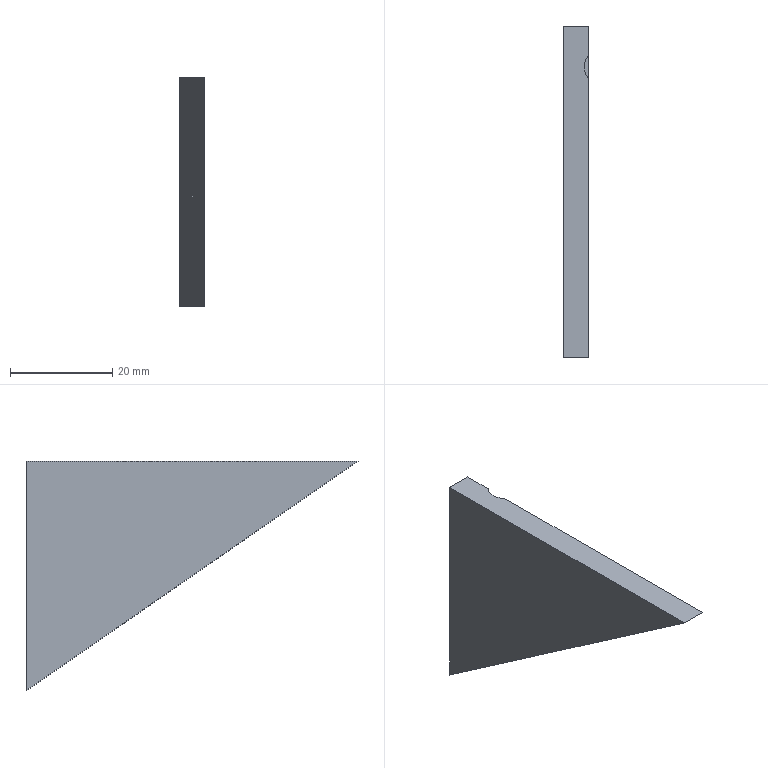Component | NX | FIXED_PLATE_14 | 1 solid | 7 faces | box 5 x 65 x 45 mm | volume 7284 mm3 | plane 6 | cylinder 1 | commonest cylinder face diameters 6.8 x1
STEP:
#1=CARTESIAN_POINT('',(0.,0.,0.));
#2=DIRECTION('',(0.,0.,1.));
#3=DIRECTION('',(1.,0.,0.));
#4=AXIS2_PLACEMENT_3D('',#1,#2,#3);
#5=CARTESIAN_POINT('',(1339.254,1356.,781.574));
#6=VERTEX_POINT('',#5);
#7=CARTESIAN_POINT('',(1339.254,1421.,736.574));
#8=VERTEX_POINT('',#7);
#9=CARTESIAN_POINT('',(1339.254,1356.,781.574));
#10=DIRECTION('',(0.,0.8222,-0.5692));
#11=VECTOR('',#10,1.);
#12=LINE('',#9,#11);
#13=CARTESIAN_POINT('',(1334.254,1356.,781.574));
#14=DIRECTION('',(0.,-0.5692,-0.8222));
#15=DIRECTION('',(0.,0.8222,-0.5692));
#16=AXIS2_PLACEMENT_3D('',#13,#14,#15);
#17=PLANE('',#16);
#18=CARTESIAN_POINT('',(0.,5.));
#19=DIRECTION('',(1.,0.));
#20=VECTOR('',#19,1.);
#21=LINE('',#18,#20);
#22=(GEOMETRIC_REPRESENTATION_CONTEXT(2)PARAMETRIC_REPRESENTATION_CONTEXT()REPRESENTATION_CONTEXT('',''));
#23=DEFINITIONAL_REPRESENTATION('',(#21),#22);
#24=PCURVE('',#17,#23);
#25=CARTESIAN_POINT('',(1339.254,0.,0.));
#26=DIRECTION('',(1.,0.,0.));
#27=DIRECTION('',(0.,0.,-1.));
#28=AXIS2_PLACEMENT_3D('',#25,#26,#27);
#29=PLANE('',#28);
#30=CARTESIAN_POINT('',(-781.574,1356.));
#31=DIRECTION('',(0.5692,0.8222));
#32=VECTOR('',#31,1.);
#33=LINE('',#30,#32);
#34=(GEOMETRIC_REPRESENTATION_CONTEXT(2)PARAMETRIC_REPRESENTATION_CONTEXT()REPRESENTATION_CONTEXT('',''));
#35=DEFINITIONAL_REPRESENTATION('',(#33),#34);
#36=PCURVE('',#29,#35);
#37=SURFACE_CURVE('',#12,(#24,#36),.PCURVE_S1.);
#38=EDGE_CURVE('',#6,#8,#37,.T.);
#39=ORIENTED_EDGE('',*,*,#38,.F.);
#40=CARTESIAN_POINT('',(1334.254,1356.,781.574));
#41=VERTEX_POINT('',#40);
#42=CARTESIAN_POINT('',(1334.254,1356.,781.574));
#43=DIRECTION('',(1.,0.,0.));
#44=VECTOR('',#43,1.);
#45=LINE('',#42,#44);
#46=CARTESIAN_POINT('',(0.,0.));
#47=DIRECTION('',(0.,1.));
#48=VECTOR('',#47,1.);
#49=LINE('',#46,#48);
#50=(GEOMETRIC_REPRESENTATION_CONTEXT(2)PARAMETRIC_REPRESENTATION_CONTEXT()REPRESENTATION_CONTEXT('',''));
#51=DEFINITIONAL_REPRESENTATION('',(#49),#50);
#52=PCURVE('',#17,#51);
#53=CARTESIAN_POINT('',(1334.254,1421.,781.574));
#54=DIRECTION('',(0.,0.,1.));
#55=DIRECTION('',(1.,0.,0.));
#56=AXIS2_PLACEMENT_3D('',#53,#54,#55);
#57=PLANE('',#56);
#58=CARTESIAN_POINT('',(0.,-65.));
#59=DIRECTION('',(1.,0.));
#60=VECTOR('',#59,1.);
#61=LINE('',#58,#60);
#62=(GEOMETRIC_REPRESENTATION_CONTEXT(2)PARAMETRIC_REPRESENTATION_CONTEXT()REPRESENTATION_CONTEXT('',''));
#63=DEFINITIONAL_REPRESENTATION('',(#61),#62);
#64=PCURVE('',#57,#63);
#65=SURFACE_CURVE('',#45,(#52,#64),.PCURVE_S1.);
#66=EDGE_CURVE('',#41,#6,#65,.T.);
#67=ORIENTED_EDGE('',*,*,#66,.F.);
#68=CARTESIAN_POINT('',(1334.254,1421.,736.574));
#69=VERTEX_POINT('',#68);
#70=CARTESIAN_POINT('',(1334.254,1356.,781.574));
#71=DIRECTION('',(0.,0.8222,-0.5692));
#72=VECTOR('',#71,1.);
#73=LINE('',#70,#72);
#74=CARTESIAN_POINT('',(0.,0.));
#75=DIRECTION('',(1.,0.));
#76=VECTOR('',#75,1.);
#77=LINE('',#74,#76);
#78=(GEOMETRIC_REPRESENTATION_CONTEXT(2)PARAMETRIC_REPRESENTATION_CONTEXT()REPRESENTATION_CONTEXT('',''));
#79=DEFINITIONAL_REPRESENTATION('',(#77),#78);
#80=PCURVE('',#17,#79);
#81=CARTESIAN_POINT('',(1334.254,0.,0.));
#82=DIRECTION('',(1.,0.,0.));
#83=DIRECTION('',(0.,0.,-1.));
#84=AXIS2_PLACEMENT_3D('',#81,#82,#83);
#85=PLANE('',#84);
#86=CARTESIAN_POINT('',(-781.574,1356.));
#87=DIRECTION('',(0.5692,0.8222));
#88=VECTOR('',#87,1.);
#89=LINE('',#86,#88);
#90=(GEOMETRIC_REPRESENTATION_CONTEXT(2)PARAMETRIC_REPRESENTATION_CONTEXT()REPRESENTATION_CONTEXT('',''));
#91=DEFINITIONAL_REPRESENTATION('',(#89),#90);
#92=PCURVE('',#85,#91);
#93=SURFACE_CURVE('',#73,(#80,#92),.PCURVE_S1.);
#94=EDGE_CURVE('',#41,#69,#93,.T.);
#95=ORIENTED_EDGE('',*,*,#94,.T.);
#96=CARTESIAN_POINT('',(1334.254,1421.,736.574));
#97=DIRECTION('',(1.,0.,0.));
#98=VECTOR('',#97,1.);
#99=LINE('',#96,#98);
#100=CARTESIAN_POINT('',(79.057,0.));
#101=DIRECTION('',(0.,1.));
#102=VECTOR('',#101,1.);
#103=LINE('',#100,#102);
#104=(GEOMETRIC_REPRESENTATION_CONTEXT(2)PARAMETRIC_REPRESENTATION_CONTEXT()REPRESENTATION_CONTEXT('',''));
#105=DEFINITIONAL_REPRESENTATION('',(#103),#104);
#106=PCURVE('',#17,#105);
#107=CARTESIAN_POINT('',(1334.254,1421.,736.574));
#108=DIRECTION('',(0.,1.,0.));
#109=DIRECTION('',(0.,0.,1.));
#110=AXIS2_PLACEMENT_3D('',#107,#108,#109);
#111=PLANE('',#110);
#112=CARTESIAN_POINT('',(0.,0.));
#113=DIRECTION('',(0.,1.));
#114=VECTOR('',#113,1.);
#115=LINE('',#112,#114);
#116=(GEOMETRIC_REPRESENTATION_CONTEXT(2)PARAMETRIC_REPRESENTATION_CONTEXT()REPRESENTATION_CONTEXT('',''));
#117=DEFINITIONAL_REPRESENTATION('',(#115),#116);
#118=PCURVE('',#111,#117);
#119=SURFACE_CURVE('',#99,(#106,#118),.PCURVE_S1.);
#120=EDGE_CURVE('',#69,#8,#119,.T.);
#121=ORIENTED_EDGE('',*,*,#120,.T.);
#122=EDGE_LOOP('',(#39,#67,#95,#121));
#123=FACE_BOUND('',#122,.T.);
#124=ADVANCED_FACE('',(#123),#17,.T.);
#125=CARTESIAN_POINT('',(1339.254,1421.,781.574));
#126=VERTEX_POINT('',#125);
#127=CARTESIAN_POINT('',(1339.254,1421.,736.574));
#128=DIRECTION('',(0.,0.,1.));
#129=VECTOR('',#128,1.);
#130=LINE('',#127,#129);
#131=CARTESIAN_POINT('',(0.,5.));
#132=DIRECTION('',(1.,0.));
#133=VECTOR('',#132,1.);
#134=LINE('',#131,#133);
#135=(GEOMETRIC_REPRESENTATION_CONTEXT(2)PARAMETRIC_REPRESENTATION_CONTEXT()REPRESENTATION_CONTEXT('',''));
#136=DEFINITIONAL_REPRESENTATION('',(#134),#135);
#137=PCURVE('',#111,#136);
#138=CARTESIAN_POINT('',(-736.574,1421.));
#139=DIRECTION('',(-1.,0.));
#140=VECTOR('',#139,1.);
#141=LINE('',#138,#140);
#142=(GEOMETRIC_REPRESENTATION_CONTEXT(2)PARAMETRIC_REPRESENTATION_CONTEXT()REPRESENTATION_CONTEXT('',''));
#143=DEFINITIONAL_REPRESENTATION('',(#141),#142);
#144=PCURVE('',#29,#143);
#145=SURFACE_CURVE('',#130,(#137,#144),.PCURVE_S1.);
#146=EDGE_CURVE('',#8,#126,#145,.T.);
#147=ORIENTED_EDGE('',*,*,#146,.F.);
#148=ORIENTED_EDGE('',*,*,#120,.F.);
#149=CARTESIAN_POINT('',(1334.254,1421.,781.574));
#150=VERTEX_POINT('',#149);
#151=CARTESIAN_POINT('',(1334.254,1421.,736.574));
#152=DIRECTION('',(0.,0.,1.));
#153=VECTOR('',#152,1.);
#154=LINE('',#151,#153);
#155=CARTESIAN_POINT('',(0.,0.));
#156=DIRECTION('',(1.,0.));
#157=VECTOR('',#156,1.);
#158=LINE('',#155,#157);
#159=(GEOMETRIC_REPRESENTATION_CONTEXT(2)PARAMETRIC_REPRESENTATION_CONTEXT()REPRESENTATION_CONTEXT('',''));
#160=DEFINITIONAL_REPRESENTATION('',(#158),#159);
#161=PCURVE('',#111,#160);
#162=CARTESIAN_POINT('',(-736.574,1421.));
#163=DIRECTION('',(-1.,0.));
#164=VECTOR('',#163,1.);
#165=LINE('',#162,#164);
#166=(GEOMETRIC_REPRESENTATION_CONTEXT(2)PARAMETRIC_REPRESENTATION_CONTEXT()REPRESENTATION_CONTEXT('',''));
#167=DEFINITIONAL_REPRESENTATION('',(#165),#166);
#168=PCURVE('',#85,#167);
#169=SURFACE_CURVE('',#154,(#161,#168),.PCURVE_S1.);
#170=EDGE_CURVE('',#69,#150,#169,.T.);
#171=ORIENTED_EDGE('',*,*,#170,.T.);
#172=CARTESIAN_POINT('',(1334.254,1421.,781.574));
#173=DIRECTION('',(1.,0.,0.));
#174=VECTOR('',#173,1.);
#175=LINE('',#172,#174);
#176=CARTESIAN_POINT('',(45.,0.));
#177=DIRECTION('',(0.,1.));
#178=VECTOR('',#177,1.);
#179=LINE('',#176,#178);
#180=(GEOMETRIC_REPRESENTATION_CONTEXT(2)PARAMETRIC_REPRESENTATION_CONTEXT()REPRESENTATION_CONTEXT('',''));
#181=DEFINITIONAL_REPRESENTATION('',(#179),#180);
#182=PCURVE('',#111,#181);
#183=CARTESIAN_POINT('',(0.,0.));
#184=DIRECTION('',(1.,0.));
#185=VECTOR('',#184,1.);
#186=LINE('',#183,#185);
#187=(GEOMETRIC_REPRESENTATION_CONTEXT(2)PARAMETRIC_REPRESENTATION_CONTEXT()REPRESENTATION_CONTEXT('',''));
#188=DEFINITIONAL_REPRESENTATION('',(#186),#187);
#189=PCURVE('',#57,#188);
#190=SURFACE_CURVE('',#175,(#182,#189),.PCURVE_S1.);
#191=EDGE_CURVE('',#150,#126,#190,.T.);
#192=ORIENTED_EDGE('',*,*,#191,.T.);
#193=EDGE_LOOP('',(#147,#148,#171,#192));
#194=FACE_BOUND('',#193,.T.);
#195=ADVANCED_FACE('',(#194),#111,.T.);
#196=CARTESIAN_POINT('',(1339.254,1415.304,781.574));
#197=VERTEX_POINT('',#196);
#198=CARTESIAN_POINT('',(1339.254,1410.696,781.574));
#199=VERTEX_POINT('',#198);
#200=CARTESIAN_POINT('',(1341.754,1413.,781.574));
#201=DIRECTION('',(0.,0.,1.));
#202=DIRECTION('',(0.,1.,0.));
#203=AXIS2_PLACEMENT_3D('',#200,#201,#202);
#204=CIRCLE('',#203,3.4);
#205=CARTESIAN_POINT('',(7.5,-8.));
#206=DIRECTION('',(0.,1.));
#207=AXIS2_PLACEMENT_2D('',#205,#206);
#208=CIRCLE('',#207,3.4);
#209=(GEOMETRIC_REPRESENTATION_CONTEXT(2)PARAMETRIC_REPRESENTATION_CONTEXT()REPRESENTATION_CONTEXT('',''));
#210=DEFINITIONAL_REPRESENTATION('',(#208),#209);
#211=PCURVE('',#57,#210);
#212=CARTESIAN_POINT('',(1341.754,1413.,771.574));
#213=DIRECTION('',(0.,0.,1.));
#214=DIRECTION('',(1.,0.,0.));
#215=AXIS2_PLACEMENT_3D('',#212,#213,#214);
#216=CYLINDRICAL_SURFACE('',#215,3.4);
#217=CARTESIAN_POINT('',(1.571,10.));
#218=DIRECTION('',(1.,0.));
#219=VECTOR('',#218,1.);
#220=LINE('',#217,#219);
#221=(GEOMETRIC_REPRESENTATION_CONTEXT(2)PARAMETRIC_REPRESENTATION_CONTEXT()REPRESENTATION_CONTEXT('',''));
#222=DEFINITIONAL_REPRESENTATION('',(#220),#221);
#223=PCURVE('',#216,#222);
#224=SURFACE_CURVE('',#204,(#211,#223),.PCURVE_S1.);
#225=EDGE_CURVE('',#197,#199,#224,.T.);
#226=ORIENTED_EDGE('',*,*,#225,.F.);
#227=CARTESIAN_POINT('',(1339.254,1421.,781.574));
#228=DIRECTION('',(0.,-1.,0.));
#229=VECTOR('',#228,1.);
#230=LINE('',#227,#229);
#231=CARTESIAN_POINT('',(5.,0.));
#232=DIRECTION('',(0.,-1.));
#233=VECTOR('',#232,1.);
#234=LINE('',#231,#233);
#235=(GEOMETRIC_REPRESENTATION_CONTEXT(2)PARAMETRIC_REPRESENTATION_CONTEXT()REPRESENTATION_CONTEXT('',''));
#236=DEFINITIONAL_REPRESENTATION('',(#234),#235);
#237=PCURVE('',#57,#236);
#238=CARTESIAN_POINT('',(-781.574,1421.));
#239=DIRECTION('',(0.,-1.));
#240=VECTOR('',#239,1.);
#241=LINE('',#238,#240);
#242=(GEOMETRIC_REPRESENTATION_CONTEXT(2)PARAMETRIC_REPRESENTATION_CONTEXT()REPRESENTATION_CONTEXT('',''));
#243=DEFINITIONAL_REPRESENTATION('',(#241),#242);
#244=PCURVE('',#29,#243);
#245=SURFACE_CURVE('',#230,(#237,#244),.PCURVE_S1.);
#246=EDGE_CURVE('',#126,#197,#245,.T.);
#247=ORIENTED_EDGE('',*,*,#246,.F.);
#248=ORIENTED_EDGE('',*,*,#191,.F.);
#249=CARTESIAN_POINT('',(1334.254,1421.,781.574));
#250=DIRECTION('',(0.,-1.,0.));
#251=VECTOR('',#250,1.);
#252=LINE('',#249,#251);
#253=CARTESIAN_POINT('',(0.,0.));
#254=DIRECTION('',(0.,-1.));
#255=VECTOR('',#254,1.);
#256=LINE('',#253,#255);
#257=(GEOMETRIC_REPRESENTATION_CONTEXT(2)PARAMETRIC_REPRESENTATION_CONTEXT()REPRESENTATION_CONTEXT('',''));
#258=DEFINITIONAL_REPRESENTATION('',(#256),#257);
#259=PCURVE('',#57,#258);
#260=CARTESIAN_POINT('',(-781.574,1421.));
#261=DIRECTION('',(0.,-1.));
#262=VECTOR('',#261,1.);
#263=LINE('',#260,#262);
#264=(GEOMETRIC_REPRESENTATION_CONTEXT(2)PARAMETRIC_REPRESENTATION_CONTEXT()REPRESENTATION_CONTEXT('',''));
#265=DEFINITIONAL_REPRESENTATION('',(#263),#264);
#266=PCURVE('',#85,#265);
#267=SURFACE_CURVE('',#252,(#259,#266),.PCURVE_S1.);
#268=EDGE_CURVE('',#150,#41,#267,.T.);
#269=ORIENTED_EDGE('',*,*,#268,.T.);
#270=ORIENTED_EDGE('',*,*,#66,.T.);
#271=CARTESIAN_POINT('',(1339.254,1421.,781.574));
#272=DIRECTION('',(0.,-1.,0.));
#273=VECTOR('',#272,1.);
#274=LINE('',#271,#273);
#275=CARTESIAN_POINT('',(5.,0.));
#276=DIRECTION('',(0.,-1.));
#277=VECTOR('',#276,1.);
#278=LINE('',#275,#277);
#279=(GEOMETRIC_REPRESENTATION_CONTEXT(2)PARAMETRIC_REPRESENTATION_CONTEXT()REPRESENTATION_CONTEXT('',''));
#280=DEFINITIONAL_REPRESENTATION('',(#278),#279);
#281=PCURVE('',#57,#280);
#282=CARTESIAN_POINT('',(-781.574,1421.));
#283=DIRECTION('',(0.,-1.));
#284=VECTOR('',#283,1.);
#285=LINE('',#282,#284);
#286=(GEOMETRIC_REPRESENTATION_CONTEXT(2)PARAMETRIC_REPRESENTATION_CONTEXT()REPRESENTATION_CONTEXT('',''));
#287=DEFINITIONAL_REPRESENTATION('',(#285),#286);
#288=PCURVE('',#29,#287);
#289=SURFACE_CURVE('',#274,(#281,#288),.PCURVE_S1.);
#290=EDGE_CURVE('',#199,#6,#289,.T.);
#291=ORIENTED_EDGE('',*,*,#290,.F.);
#292=EDGE_LOOP('',(#226,#247,#248,#269,#270,#291));
#293=FACE_BOUND('',#292,.T.);
#294=ADVANCED_FACE('',(#293),#57,.T.);
#295=ORIENTED_EDGE('',*,*,#94,.F.);
#296=ORIENTED_EDGE('',*,*,#268,.F.);
#297=ORIENTED_EDGE('',*,*,#170,.F.);
#298=EDGE_LOOP('',(#295,#296,#297));
#299=FACE_BOUND('',#298,.T.);
#300=ADVANCED_FACE('',(#299),#85,.F.);
#301=CARTESIAN_POINT('',(1339.254,1415.304,771.574));
#302=VERTEX_POINT('',#301);
#303=CARTESIAN_POINT('',(1339.254,1415.304,771.574));
#304=DIRECTION('',(0.,0.,1.));
#305=VECTOR('',#304,1.);
#306=LINE('',#303,#305);
#307=CARTESIAN_POINT('',(-771.574,1415.304));
#308=DIRECTION('',(-1.,0.));
#309=VECTOR('',#308,1.);
#310=LINE('',#307,#309);
#311=(GEOMETRIC_REPRESENTATION_CONTEXT(2)PARAMETRIC_REPRESENTATION_CONTEXT()REPRESENTATION_CONTEXT('',''));
#312=DEFINITIONAL_REPRESENTATION('',(#310),#311);
#313=PCURVE('',#29,#312);
#314=CARTESIAN_POINT('',(2.397,0.));
#315=DIRECTION('',(0.,1.));
#316=VECTOR('',#315,1.);
#317=LINE('',#314,#316);
#318=(GEOMETRIC_REPRESENTATION_CONTEXT(2)PARAMETRIC_REPRESENTATION_CONTEXT()REPRESENTATION_CONTEXT('',''));
#319=DEFINITIONAL_REPRESENTATION('',(#317),#318);
#320=PCURVE('',#216,#319);
#321=SURFACE_CURVE('',#306,(#313,#320),.PCURVE_S1.);
#322=EDGE_CURVE('',#302,#197,#321,.T.);
#323=ORIENTED_EDGE('',*,*,#322,.F.);
#324=CARTESIAN_POINT('',(1339.254,1410.696,771.574));
#325=VERTEX_POINT('',#324);
#326=CARTESIAN_POINT('',(1339.254,0.,771.574));
#327=DIRECTION('',(0.,-1.,0.));
#328=VECTOR('',#327,1.);
#329=LINE('',#326,#328);
#330=CARTESIAN_POINT('',(-771.574,0.));
#331=DIRECTION('',(0.,-1.));
#332=VECTOR('',#331,1.);
#333=LINE('',#330,#332);
#334=(GEOMETRIC_REPRESENTATION_CONTEXT(2)PARAMETRIC_REPRESENTATION_CONTEXT()REPRESENTATION_CONTEXT('',''));
#335=DEFINITIONAL_REPRESENTATION('',(#333),#334);
#336=PCURVE('',#29,#335);
#337=CARTESIAN_POINT('',(1341.754,1413.,771.574));
#338=DIRECTION('',(0.,0.,1.));
#339=DIRECTION('',(1.,0.,0.));
#340=AXIS2_PLACEMENT_3D('',#337,#338,#339);
#341=PLANE('',#340);
#342=CARTESIAN_POINT('',(-2.5,-1413.));
#343=DIRECTION('',(0.,-1.));
#344=VECTOR('',#343,1.);
#345=LINE('',#342,#344);
#346=(GEOMETRIC_REPRESENTATION_CONTEXT(2)PARAMETRIC_REPRESENTATION_CONTEXT()REPRESENTATION_CONTEXT('',''));
#347=DEFINITIONAL_REPRESENTATION('',(#345),#346);
#348=PCURVE('',#341,#347);
#349=SURFACE_CURVE('',#329,(#336,#348),.PCURVE_S1.);
#350=EDGE_CURVE('',#302,#325,#349,.T.);
#351=ORIENTED_EDGE('',*,*,#350,.T.);
#352=CARTESIAN_POINT('',(1339.254,1410.696,771.574));
#353=DIRECTION('',(0.,0.,-1.));
#354=VECTOR('',#353,1.);
#355=LINE('',#352,#354);
#356=CARTESIAN_POINT('',(-771.574,1410.696));
#357=DIRECTION('',(1.,0.));
#358=VECTOR('',#357,1.);
#359=LINE('',#356,#358);
#360=(GEOMETRIC_REPRESENTATION_CONTEXT(2)PARAMETRIC_REPRESENTATION_CONTEXT()REPRESENTATION_CONTEXT('',''));
#361=DEFINITIONAL_REPRESENTATION('',(#359),#360);
#362=PCURVE('',#29,#361);
#363=CARTESIAN_POINT('',(3.886,0.));
#364=DIRECTION('',(0.,-1.));
#365=VECTOR('',#364,1.);
#366=LINE('',#363,#365);
#367=(GEOMETRIC_REPRESENTATION_CONTEXT(2)PARAMETRIC_REPRESENTATION_CONTEXT()REPRESENTATION_CONTEXT('',''));
#368=DEFINITIONAL_REPRESENTATION('',(#366),#367);
#369=PCURVE('',#216,#368);
#370=SURFACE_CURVE('',#355,(#362,#369),.PCURVE_S1.);
#371=EDGE_CURVE('',#199,#325,#370,.T.);
#372=ORIENTED_EDGE('',*,*,#371,.F.);
#373=ORIENTED_EDGE('',*,*,#290,.T.);
#374=ORIENTED_EDGE('',*,*,#38,.T.);
#375=ORIENTED_EDGE('',*,*,#146,.T.);
#376=ORIENTED_EDGE('',*,*,#246,.T.);
#377=EDGE_LOOP('',(#323,#351,#372,#373,#374,#375,#376));
#378=FACE_BOUND('',#377,.T.);
#379=ADVANCED_FACE('',(#378),#29,.T.);
#380=CARTESIAN_POINT('',(1341.754,1413.,771.574));
#381=DIRECTION('',(0.,0.,-1.));
#382=DIRECTION('',(0.,1.,0.));
#383=AXIS2_PLACEMENT_3D('',#380,#381,#382);
#384=CIRCLE('',#383,3.4);
#385=CARTESIAN_POINT('',(7.854,0.));
#386=DIRECTION('',(-1.,0.));
#387=VECTOR('',#386,1.);
#388=LINE('',#385,#387);
#389=(GEOMETRIC_REPRESENTATION_CONTEXT(2)PARAMETRIC_REPRESENTATION_CONTEXT()REPRESENTATION_CONTEXT('',''));
#390=DEFINITIONAL_REPRESENTATION('',(#388),#389);
#391=PCURVE('',#216,#390);
#392=CARTESIAN_POINT('',(0.,3.4));
#393=CARTESIAN_POINT('',(5.889,3.4));
#394=CARTESIAN_POINT('',(2.944,-1.7));
#395=CARTESIAN_POINT('',(0.,-6.8));
#396=CARTESIAN_POINT('',(-2.944,-1.7));
#397=CARTESIAN_POINT('',(-5.889,3.4));
#398=CARTESIAN_POINT('',(0.,3.4));
#399=(BOUNDED_CURVE()B_SPLINE_CURVE(2,(#392,#393,#394,#395,#396,#397,#398),.UNSPECIFIED.,.T.,.F.)B_SPLINE_CURVE_WITH_KNOTS((1,2,2,2,2,1),(-2.094,0.,2.094,4.189,6.283,8.378),.UNSPECIFIED.)CURVE()GEOMETRIC_REPRESENTATION_ITEM()RATIONAL_B_SPLINE_CURVE((1.,0.5,1.,0.5,1.,0.5,1.))REPRESENTATION_ITEM(''));
#400=(GEOMETRIC_REPRESENTATION_CONTEXT(2)PARAMETRIC_REPRESENTATION_CONTEXT()REPRESENTATION_CONTEXT('',''));
#401=DEFINITIONAL_REPRESENTATION('',(#399),#400);
#402=PCURVE('',#341,#401);
#403=SURFACE_CURVE('',#384,(#391,#402),.PCURVE_S1.);
#404=EDGE_CURVE('',#325,#302,#403,.T.);
#405=ORIENTED_EDGE('',*,*,#404,.F.);
#406=ORIENTED_EDGE('',*,*,#371,.F.);
#407=ORIENTED_EDGE('',*,*,#225,.F.);
#408=ORIENTED_EDGE('',*,*,#322,.F.);
#409=EDGE_LOOP('',(#405,#406,#407,#408));
#410=FACE_BOUND('',#409,.F.);
#411=ADVANCED_FACE('',(#410),#216,.F.);
#412=ORIENTED_EDGE('',*,*,#404,.F.);
#413=ORIENTED_EDGE('',*,*,#350,.F.);
#414=EDGE_LOOP('',(#412,#413));
#415=FACE_BOUND('',#414,.T.);
#416=ADVANCED_FACE('',(#415),#341,.T.);
#417=CLOSED_SHELL('',(#124,#195,#294,#300,#379,#411,#416));
#418=MANIFOLD_SOLID_BREP('',#417);
#419=(LENGTH_UNIT()NAMED_UNIT(*)SI_UNIT(.MILLI.,.METRE.));
#420=UNCERTAINTY_MEASURE_WITH_UNIT(LENGTH_MEASURE(0.0000001),#419,'','');
#421=(NAMED_UNIT(*)PLANE_ANGLE_UNIT()SI_UNIT($,.RADIAN.));
#422=(NAMED_UNIT(*)SI_UNIT($,.STERADIAN.)SOLID_ANGLE_UNIT());
#423=(GEOMETRIC_REPRESENTATION_CONTEXT(3)GLOBAL_UNCERTAINTY_ASSIGNED_CONTEXT((#420))GLOBAL_UNIT_ASSIGNED_CONTEXT((#419,#421,#422))REPRESENTATION_CONTEXT('',''));
#424=ADVANCED_BREP_SHAPE_REPRESENTATION('',(#4,#418),#423);